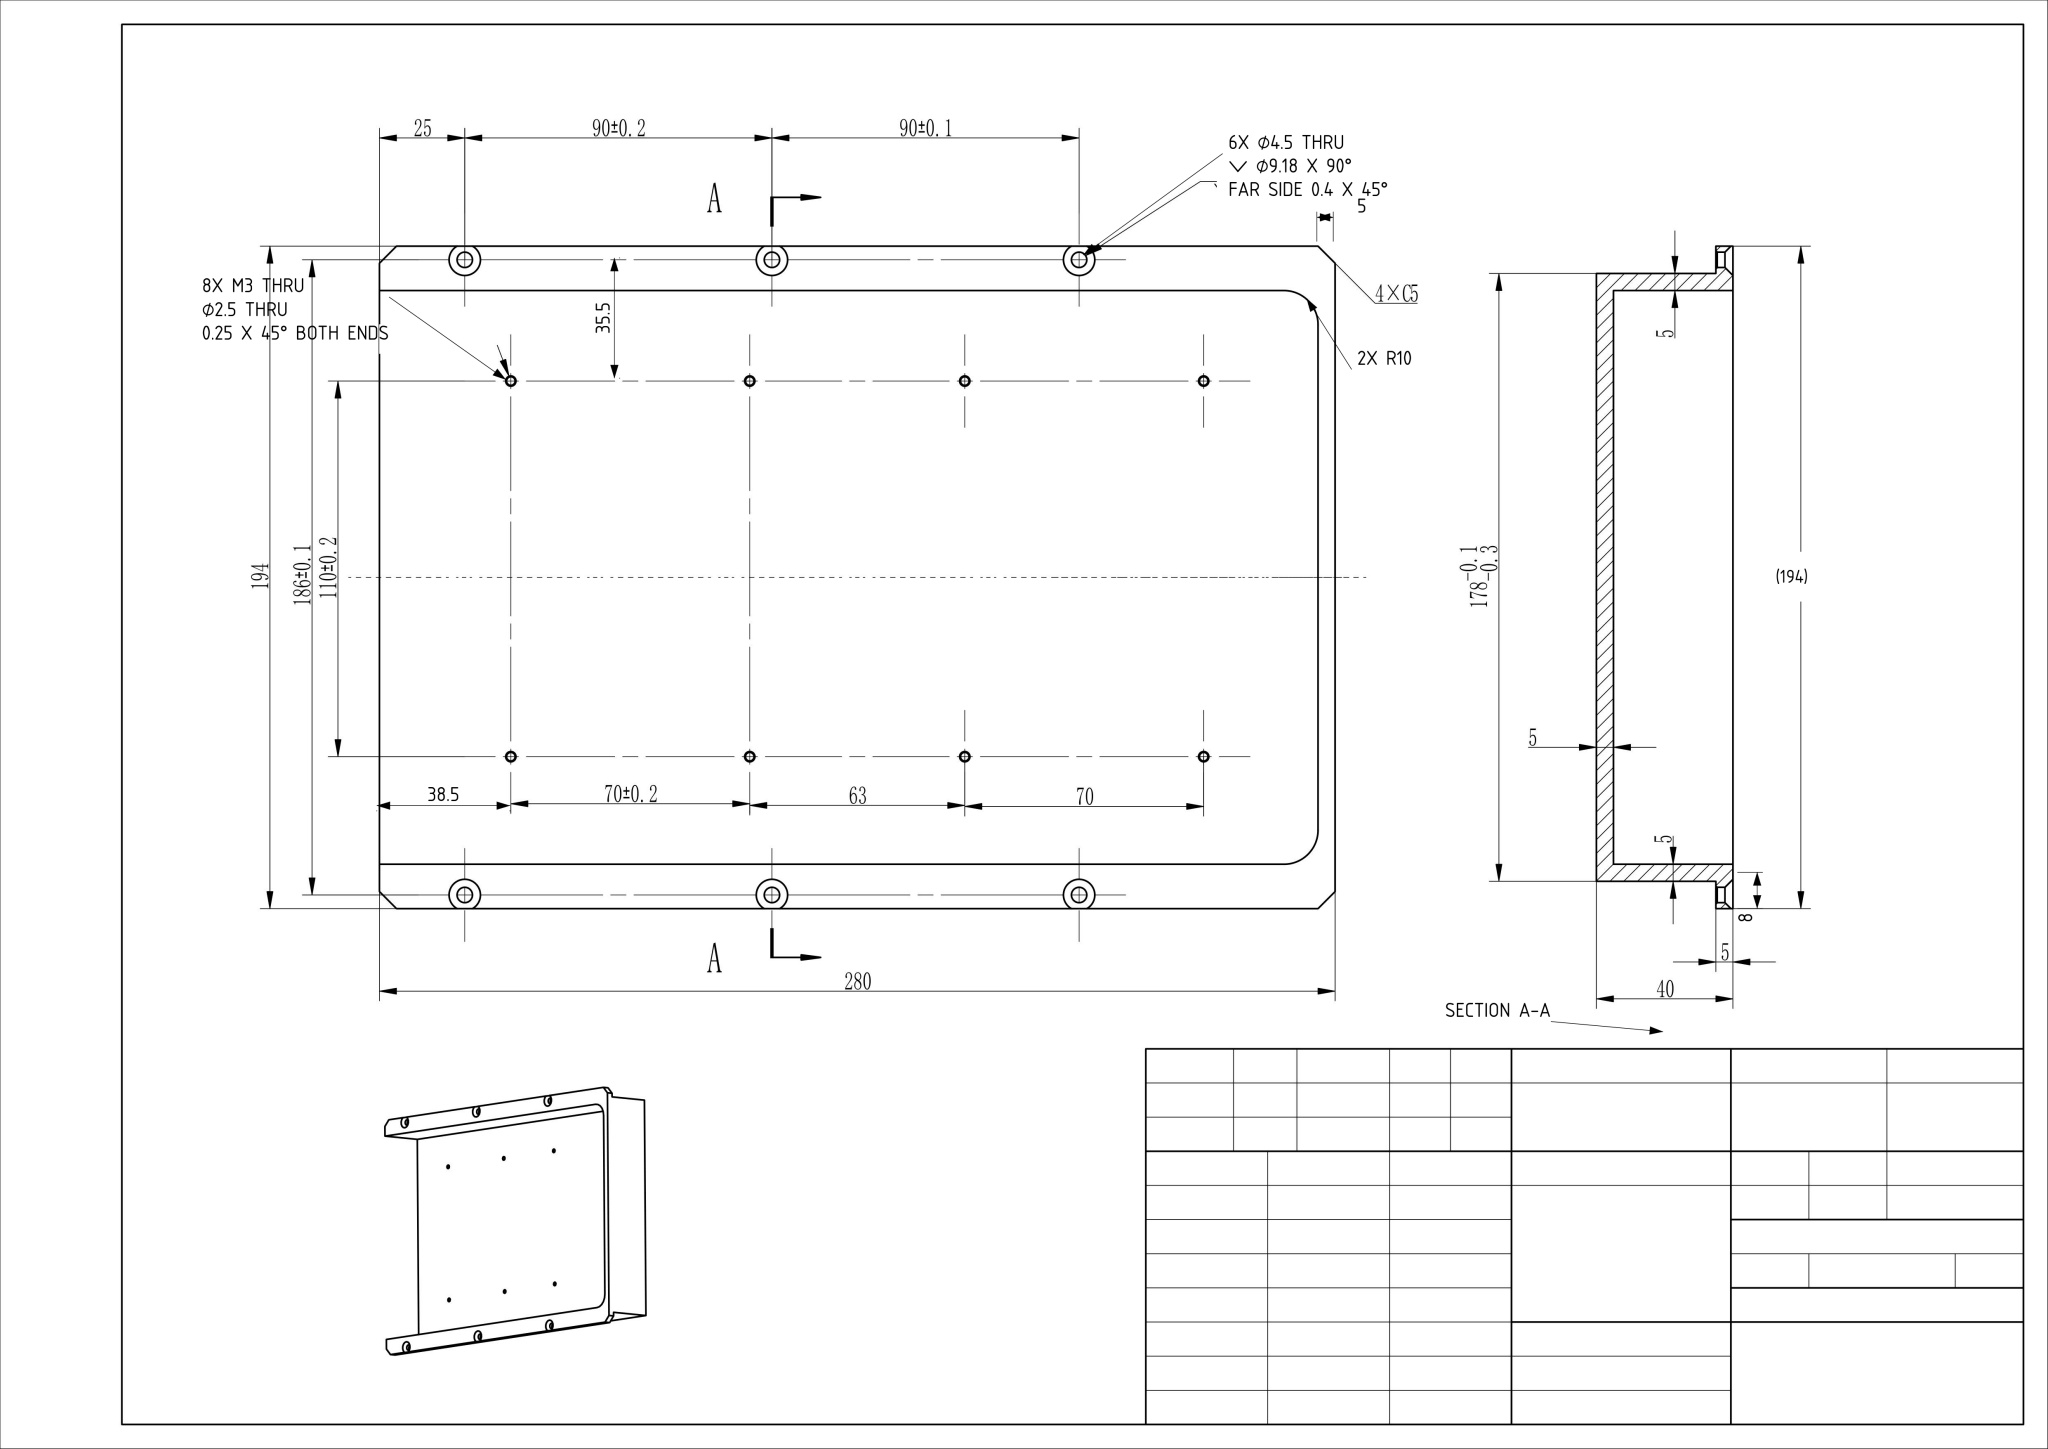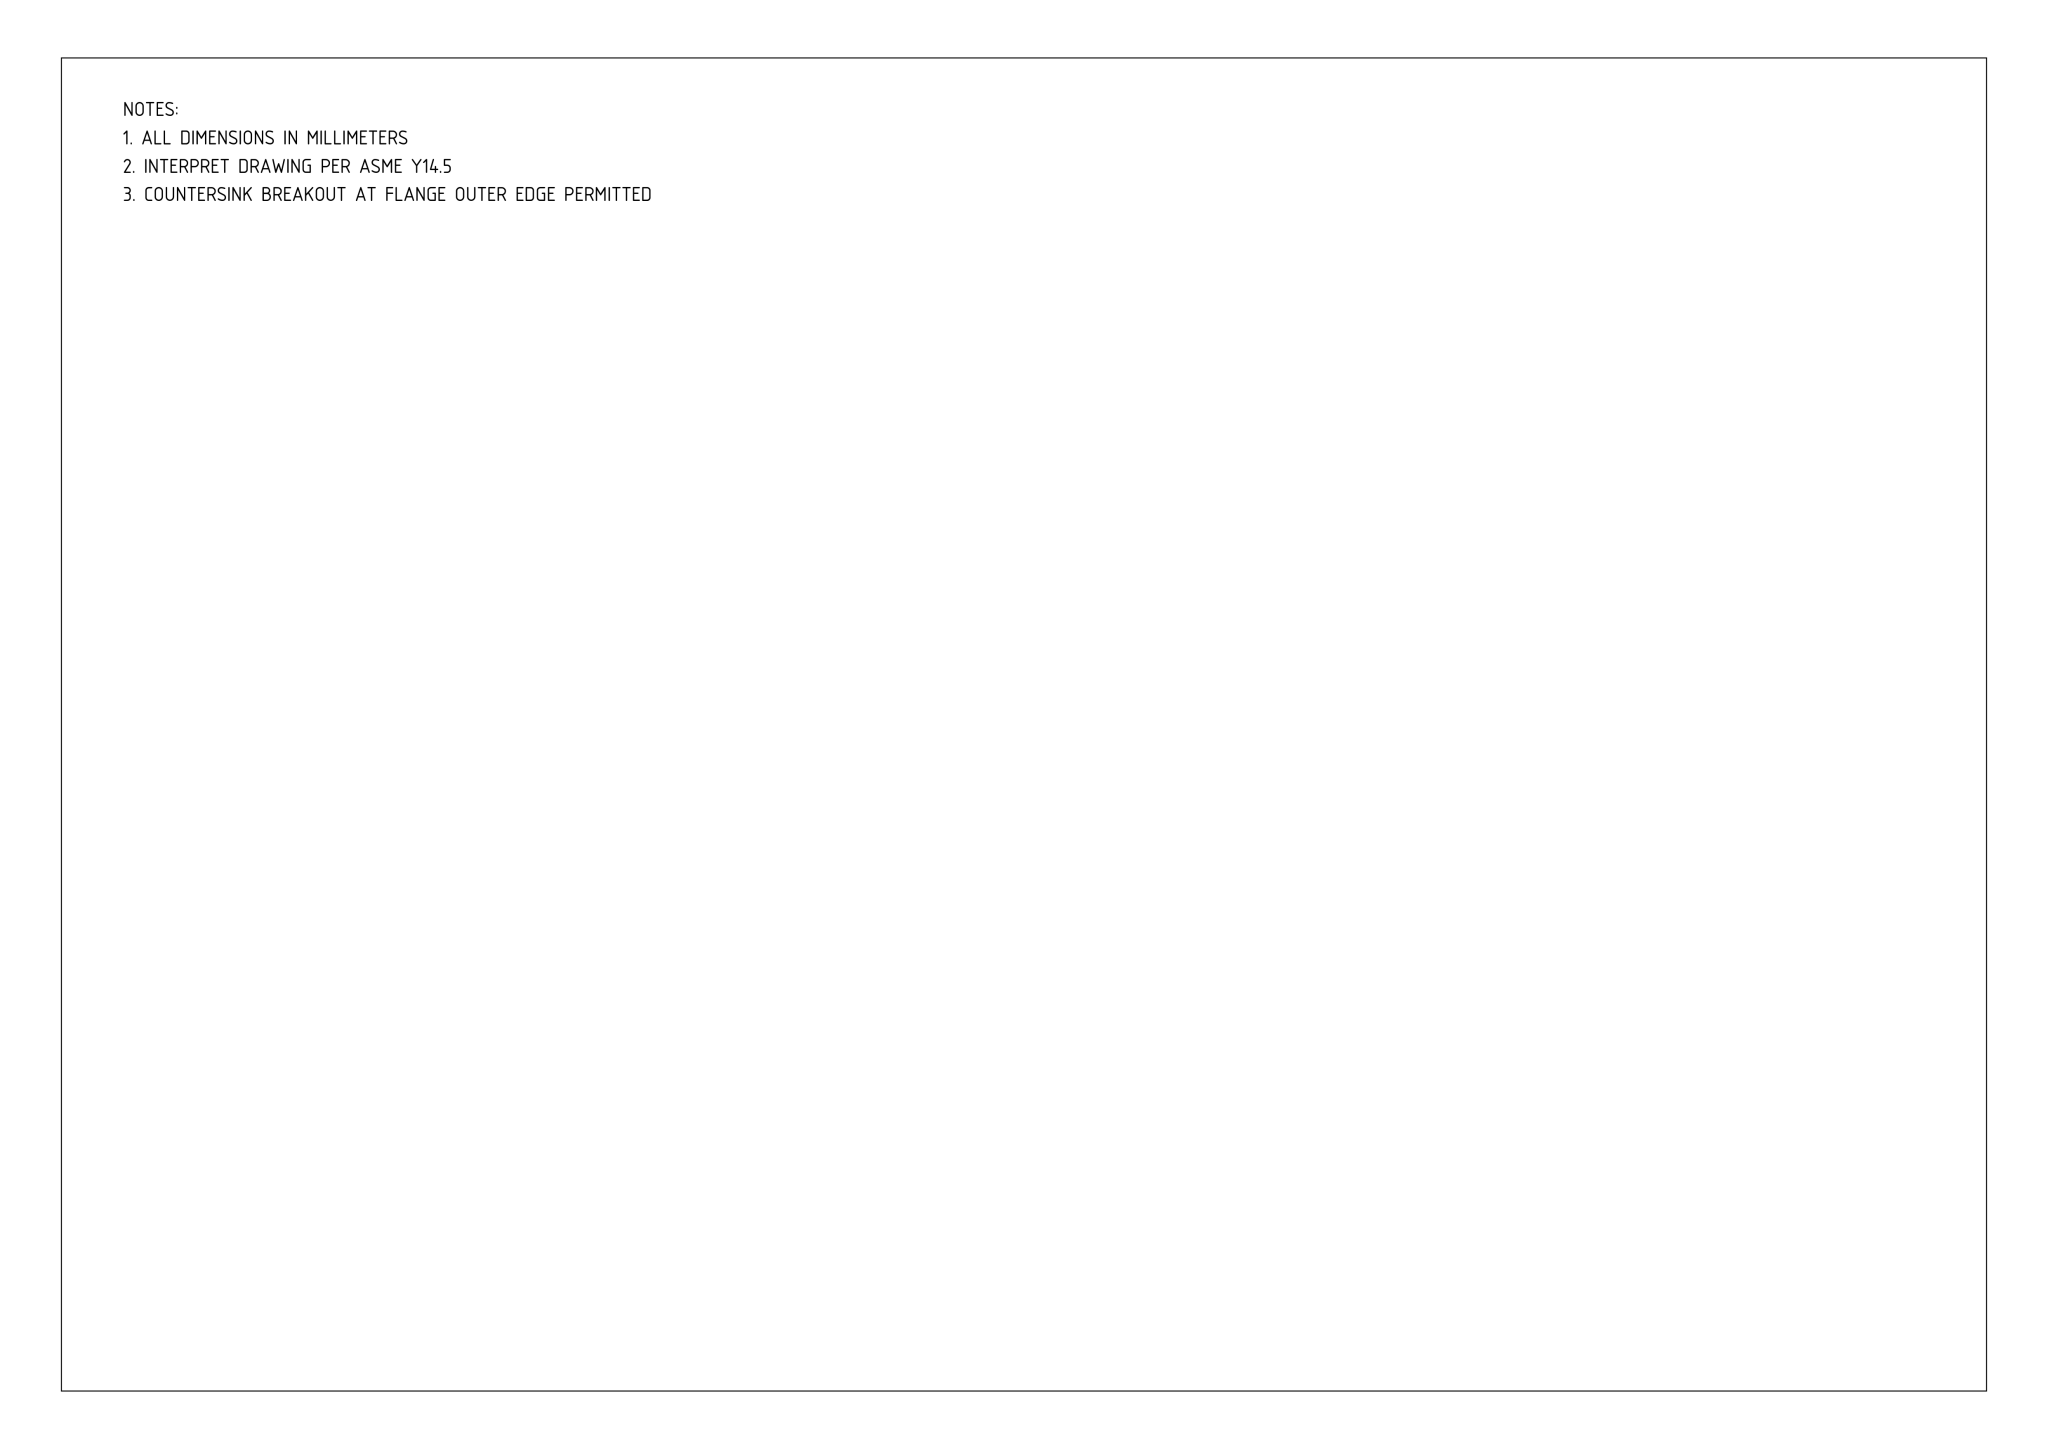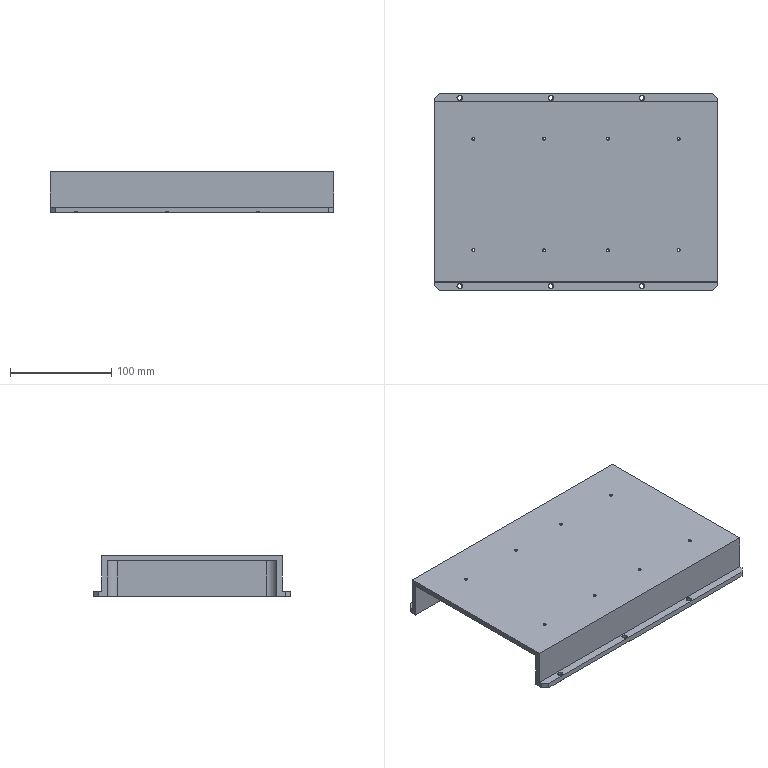Part | NX | mm | 1 solid | 62 faces | box 280 x 194 x 40 mm | volume 399257 mm3 | cone 28 | plane 18 | cylinder 16 | commonest cylinder face diameters 2.5 x8 4.5 x6 20 x2